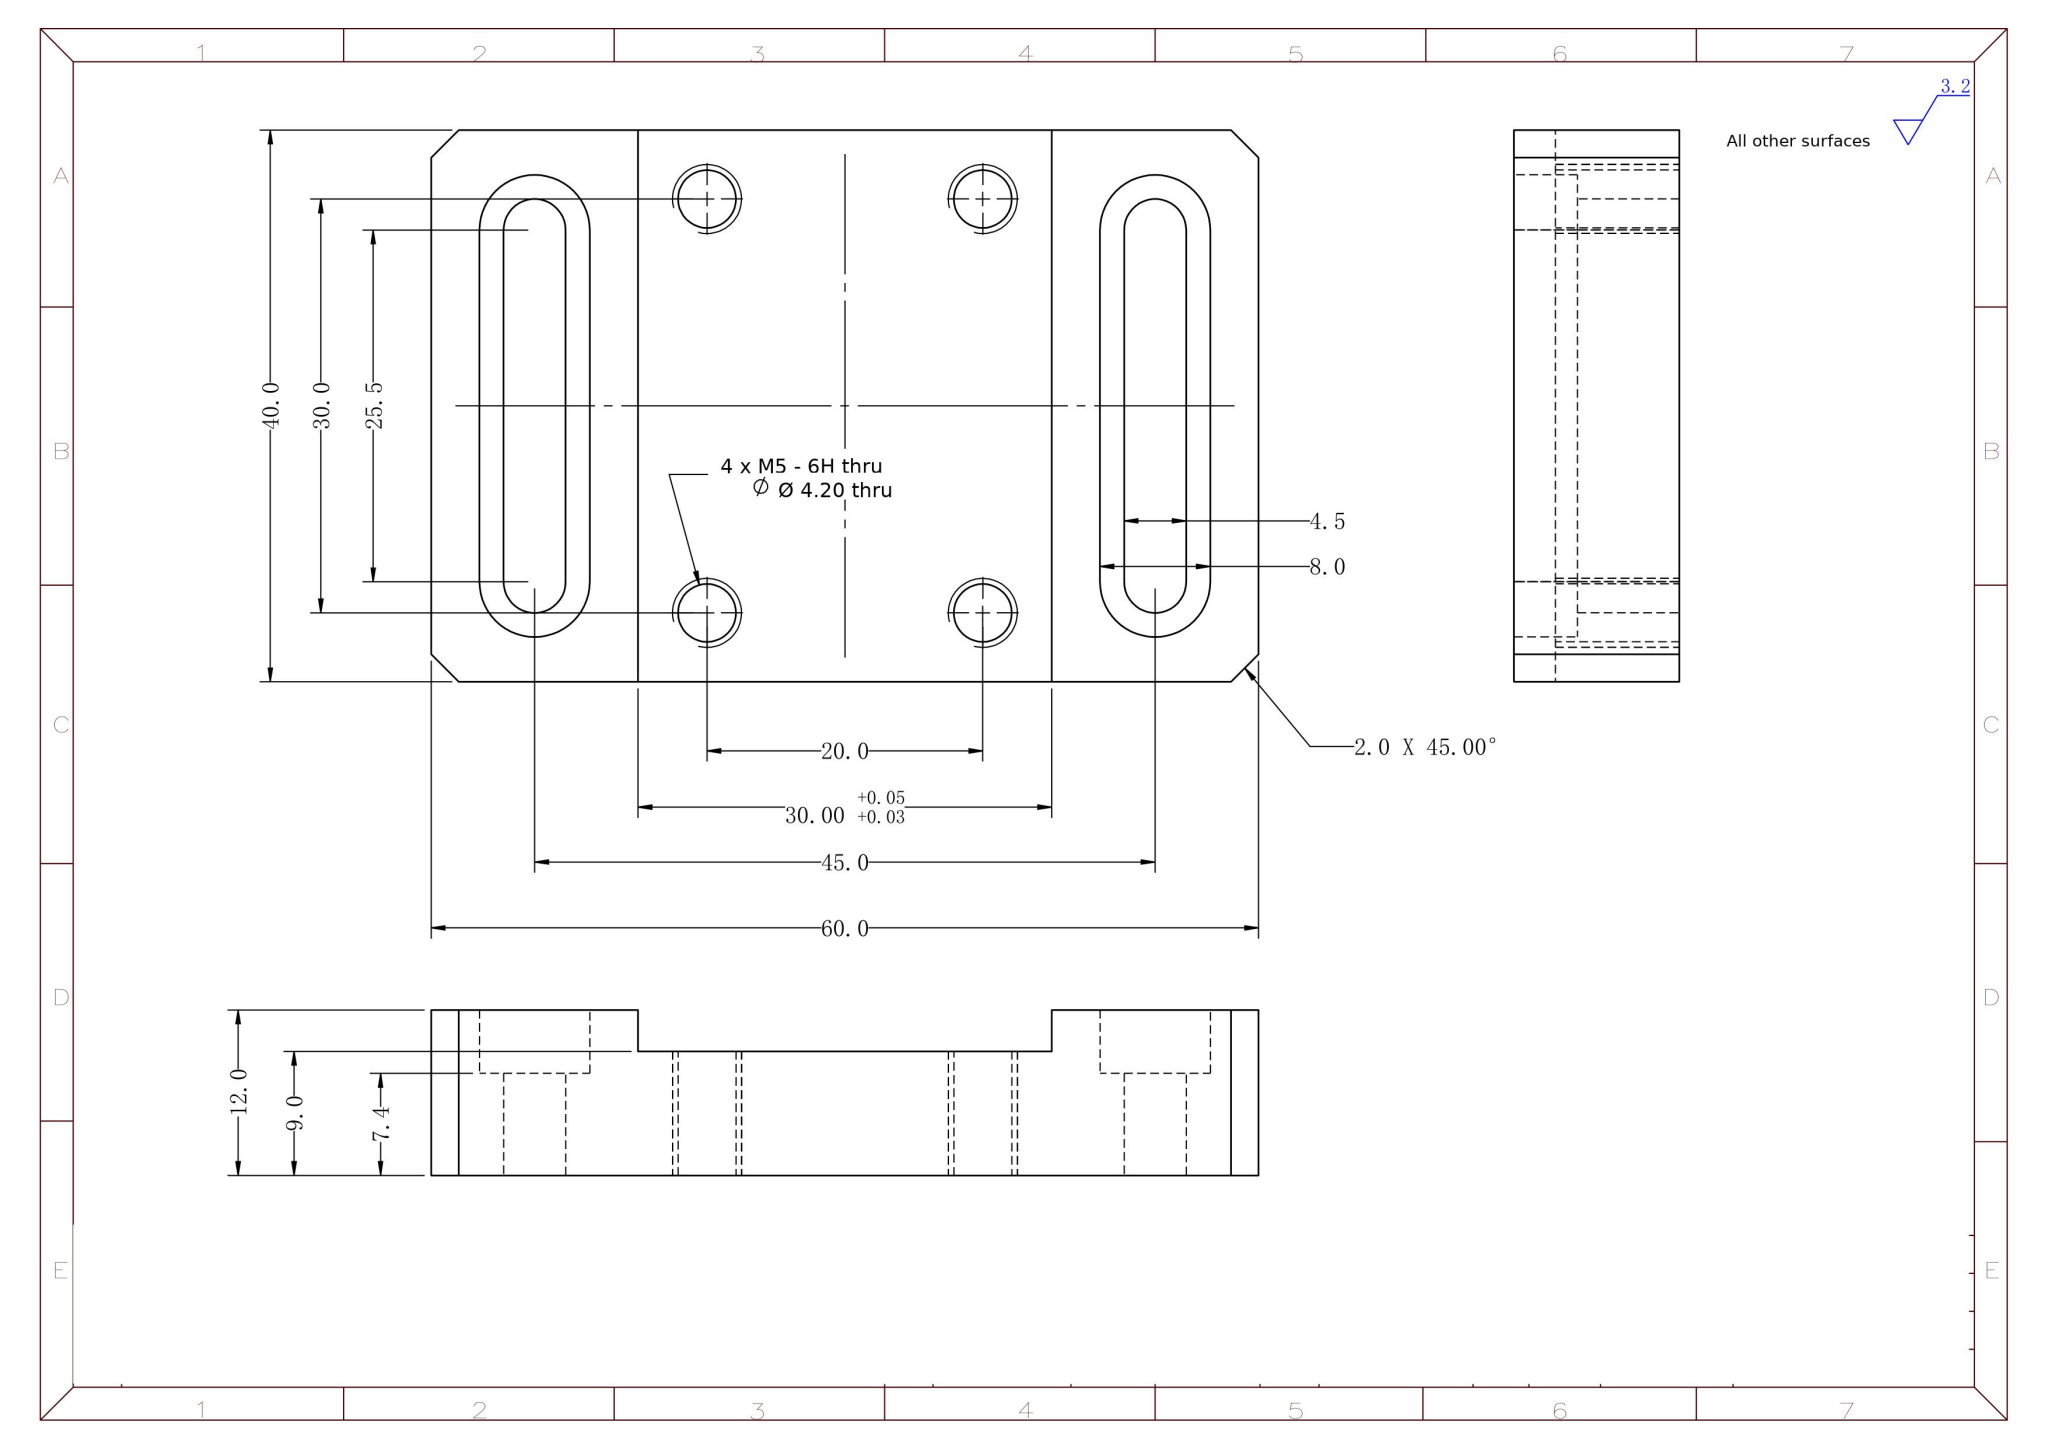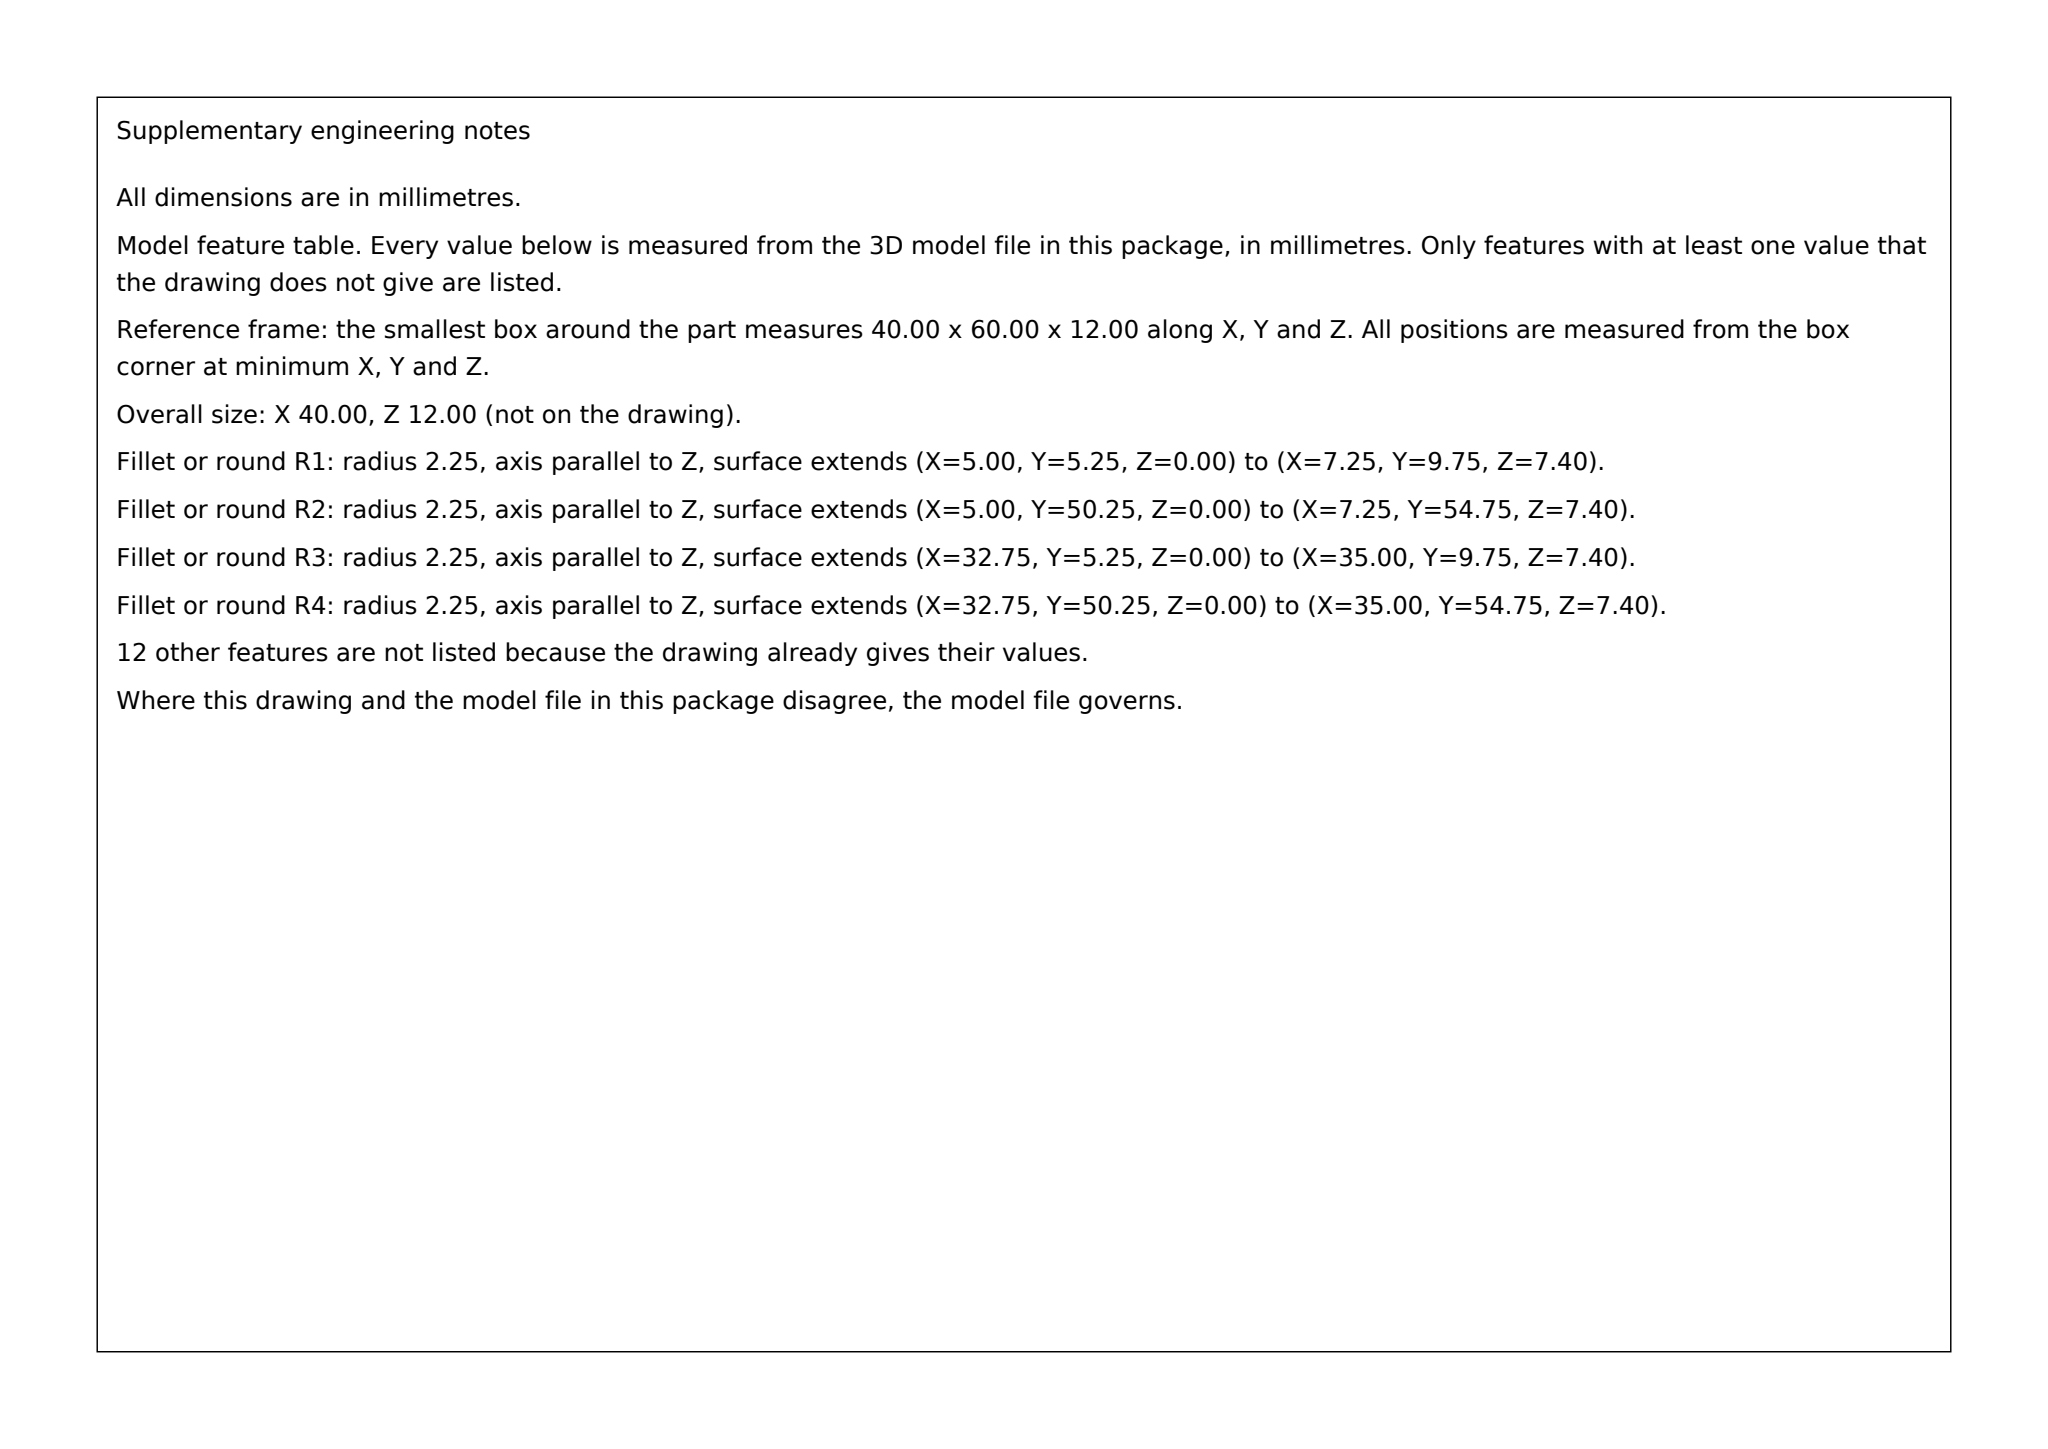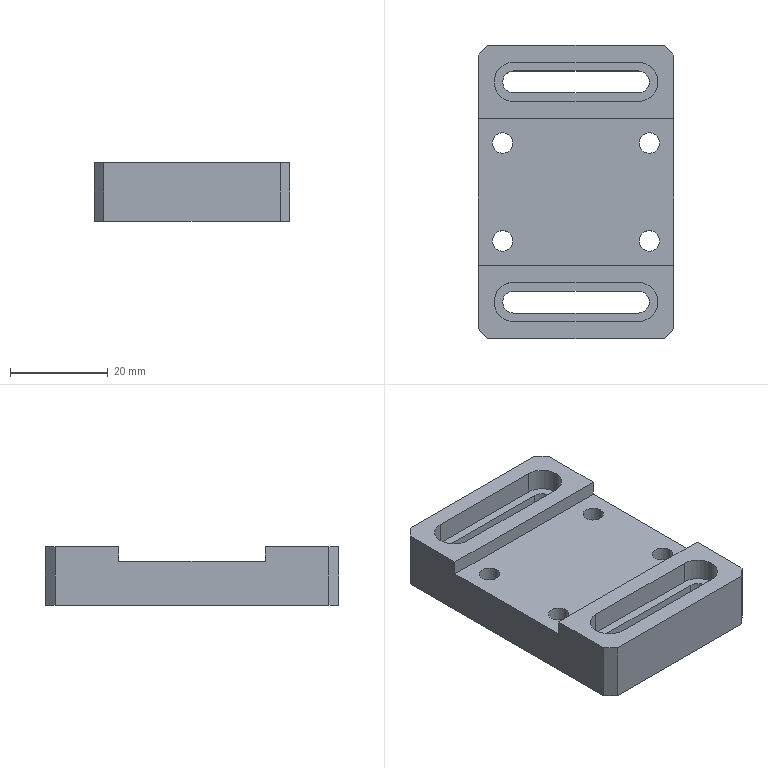Part | SolidWorks | mm | 1 solid | 44 faces | box 40 x 60 x 12 mm | volume 20332 mm3 | plane 24 | cylinder 20 | commonest cylinder face diameters 4.2 x8 8 x6 4.5 x6